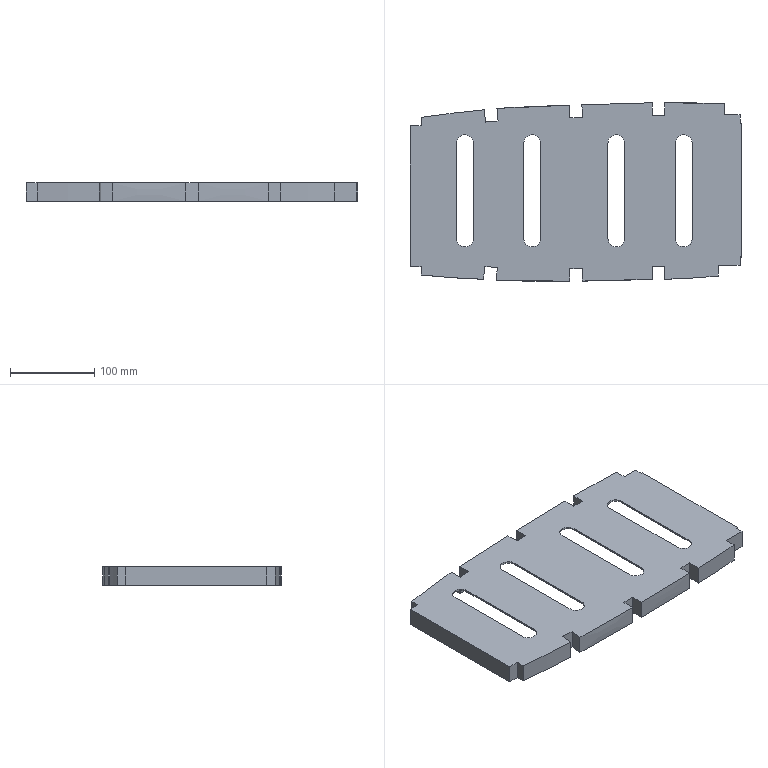Component | NX | MID_RIB_4 | 1 solid | 99 faces | volume 190356 mm3 | plane 75 | cylinder 8 | other 8 | spline 8 | commonest cylinder face diameters 20 x8